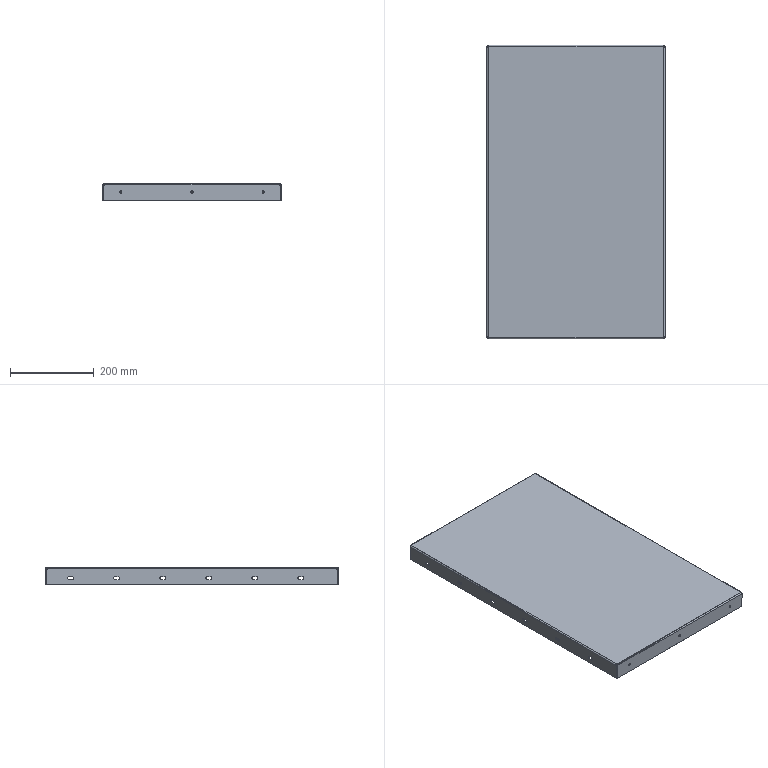Component | SolidWorks | DrawerAssembly-1_Drawer-1 | 1 solid | 128 faces | volume 758526 mm3 | plane 78 | cylinder 50 | commonest cylinder face diameters 7 x36 5 x6 6 x4 2 x4